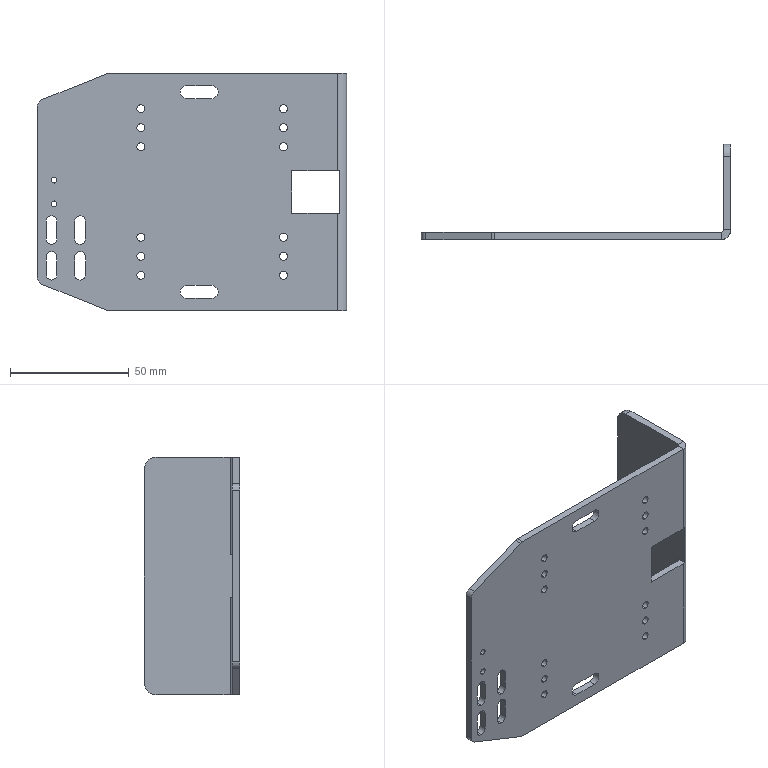Component | SolidWorks | XM-02-005A1-1 | 1 solid | 82 faces | volume 46156 mm3 | cylinder 53 | plane 29 | commonest cylinder face diameters 3.3 x24 4.5 x12 2.5 x4 5.5 x4 6 x4 2 x2 10 x2 8 x1 | material SUS304